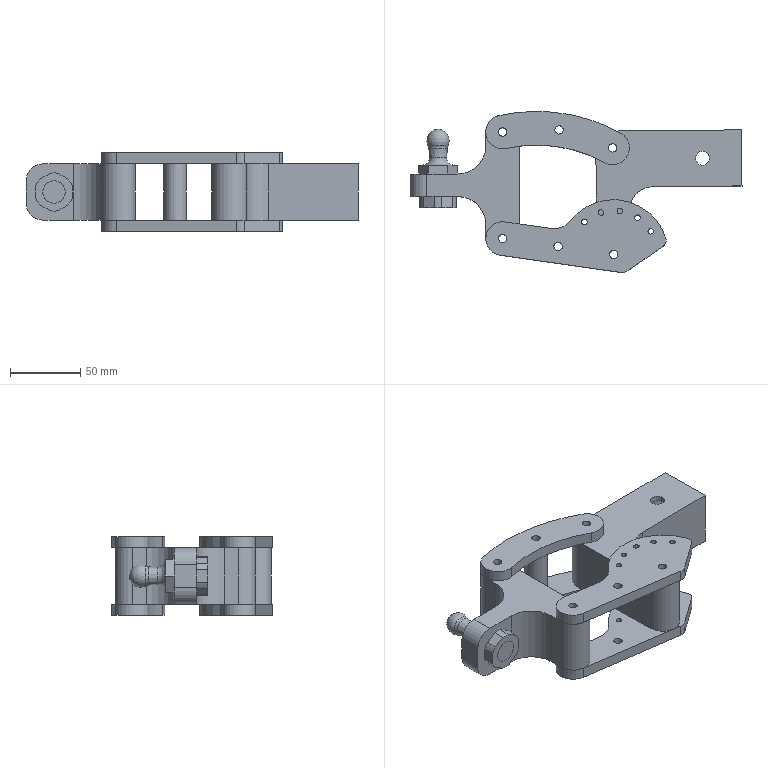Assembly | NX | mm | 9 component files | 9 solids | 124 faces | box 236.81 x 114.89 x 56 mm | volume 417923 mm3 | cylinder 67 | plane 53 | torus 2 | cone 1 | sphere 1 | commonest cylinder face diameters 6 x17 24 x11 4 x11 16 x6 27.34 x6 10 x4 40 x2 199.98 x2
Bill of materials:
unnamed part 1 | 1 |  | Curved, banana-shaped flat plate of uniform thickness with fully rounded ends and three round through-holes spaced along the arc.
unnamed part 2 | 1 |  | Turned pin-like part with a plain cylindrical shank, a hexagonal collar, and a short neck that flares at the collar, narrows, and ends in a spherical ball.
unnamed part 3 | 1 |  | Flat plate of uniform thickness with an irregular outline: a straight arm with a rounded end that widens into a large rounded lobe. It has three larger through-holes and five smaller through-holes arranged on an arc in the lobe.
unnamed part 4 | 1 |  | T-shaped block: a thick bar with rounded ends, each end with a small vertical through-hole. A thinner perpendicular tab with a rounded end extends from the middle of the bar and is joined to it by large concave fillets. The tab has one large through-hole running across its thickness.
unnamed part 5 | 1 |  | Flat plate of uniform thickness with an arm that widens into a large rounded lobe. It has three larger through-holes and five smaller through-holes on an arc in the lobe.
unnamed part 6 | 1 |  | Plain cylindrical tube or sleeve with a concentric round through-bore and flat ends. Its length is roughly 2.5 times its outer diameter.
unnamed part 7 | 1 |  | Curved, arc-shaped flat plate of uniform thickness with rounded ends and three round through-holes along its length.
unnamed part 8 | 1 |  | L-shaped block of constant height. One leg ends in a rounded end; the other has square-cut ends and appears to be hollow, with a thin-walled rectangular opening at its end face. The inside corner is filleted. The top face has four round holes of different sizes.
unnamed part 9 | 1 |  | Short ring-shaped part with a large central round bore. Its outer profile is a hexagon with the corners trimmed by arcs, so six flat faces alternate with rounded corners. Its thickness is small compared with its width.
Mates:
1. slider | 6 1 face | 6 1 point | front_bracket 1 face | front_bracket 1 point
2. touch align | 6 1 face | front_bracket 1 face
3. fix | front_bracket 1 component
4. concentric | 7 1 edge | front_bracket 1 edge
5. concentric | 3 1 edge | front_bracket 1 edge
6. concentric | 5 1 edge | 3 1 edge
7. concentric | 4 1 edge | front_bracket 1 edge
8. concentric | 4 1 edge | 5 1 edge
9. concentric | 2 1 edge | 4 1 edge